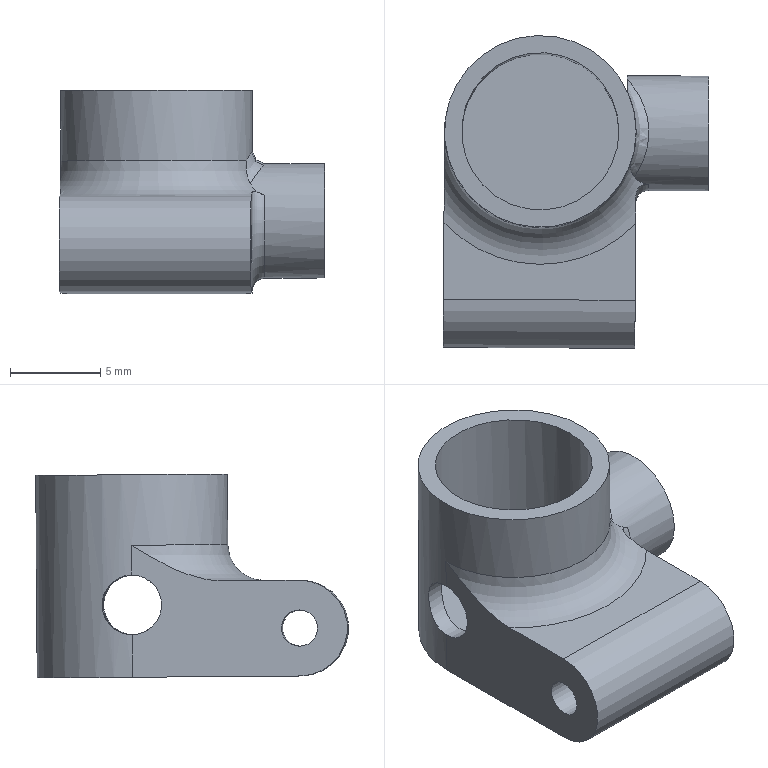Component | NX | SUPPORT | 1 solid | 19 faces | volume 921 mm3 | plane 8 | cylinder 7 | torus 2 | spline 2 | commonest cylinder face diameters 3.3 x2 10.6 x1 5.3 x1 8.7 x1 6.35 x1 2 x1